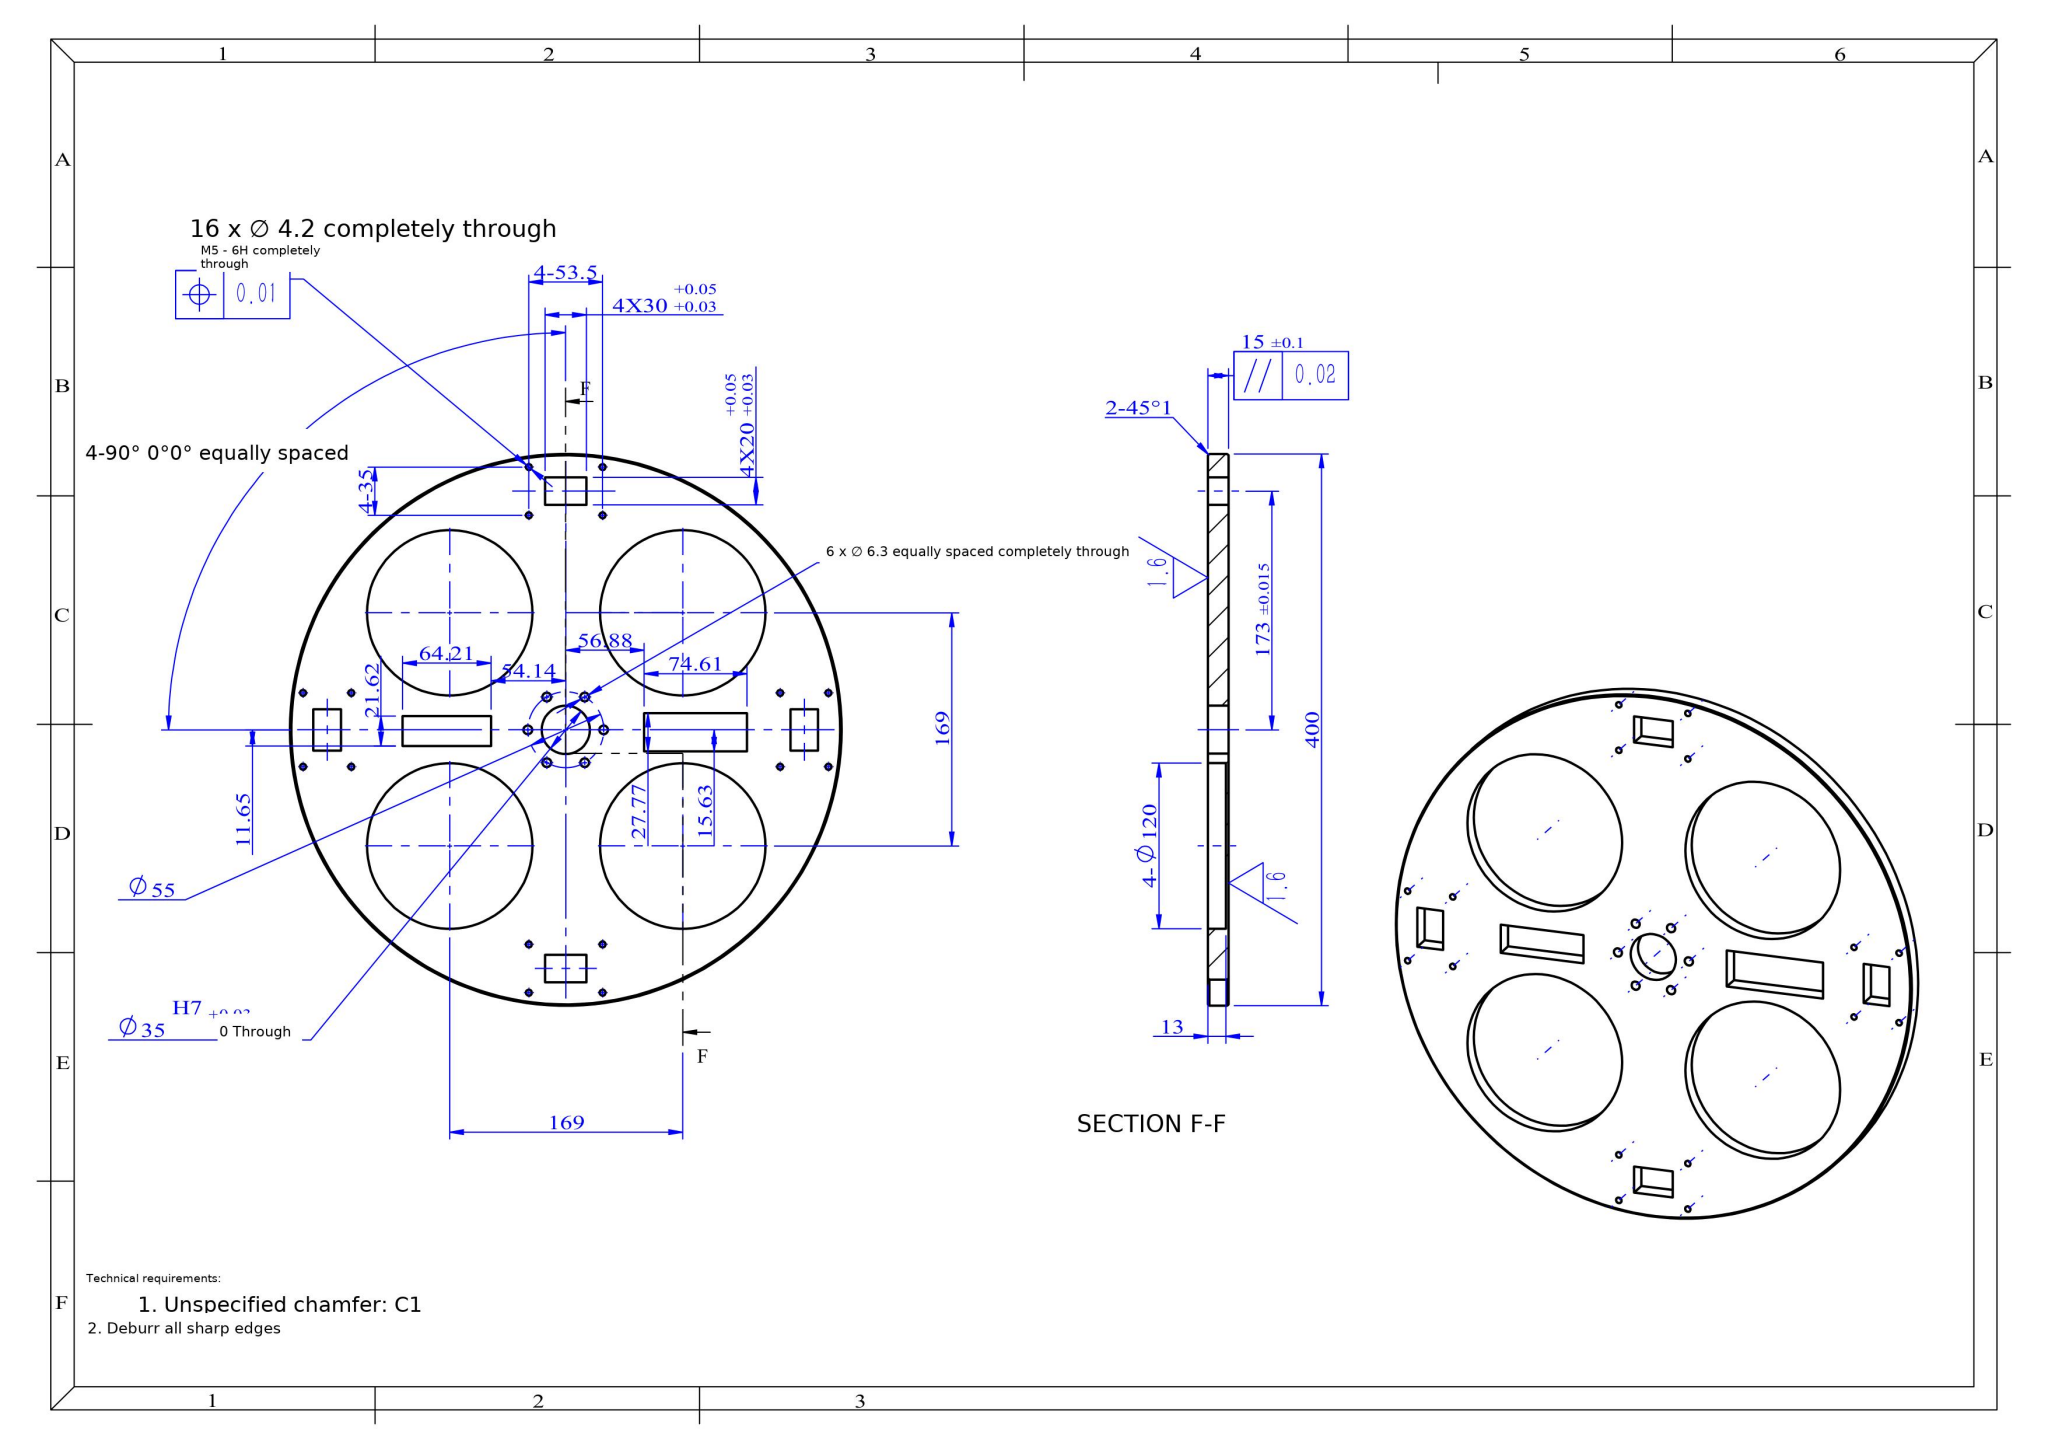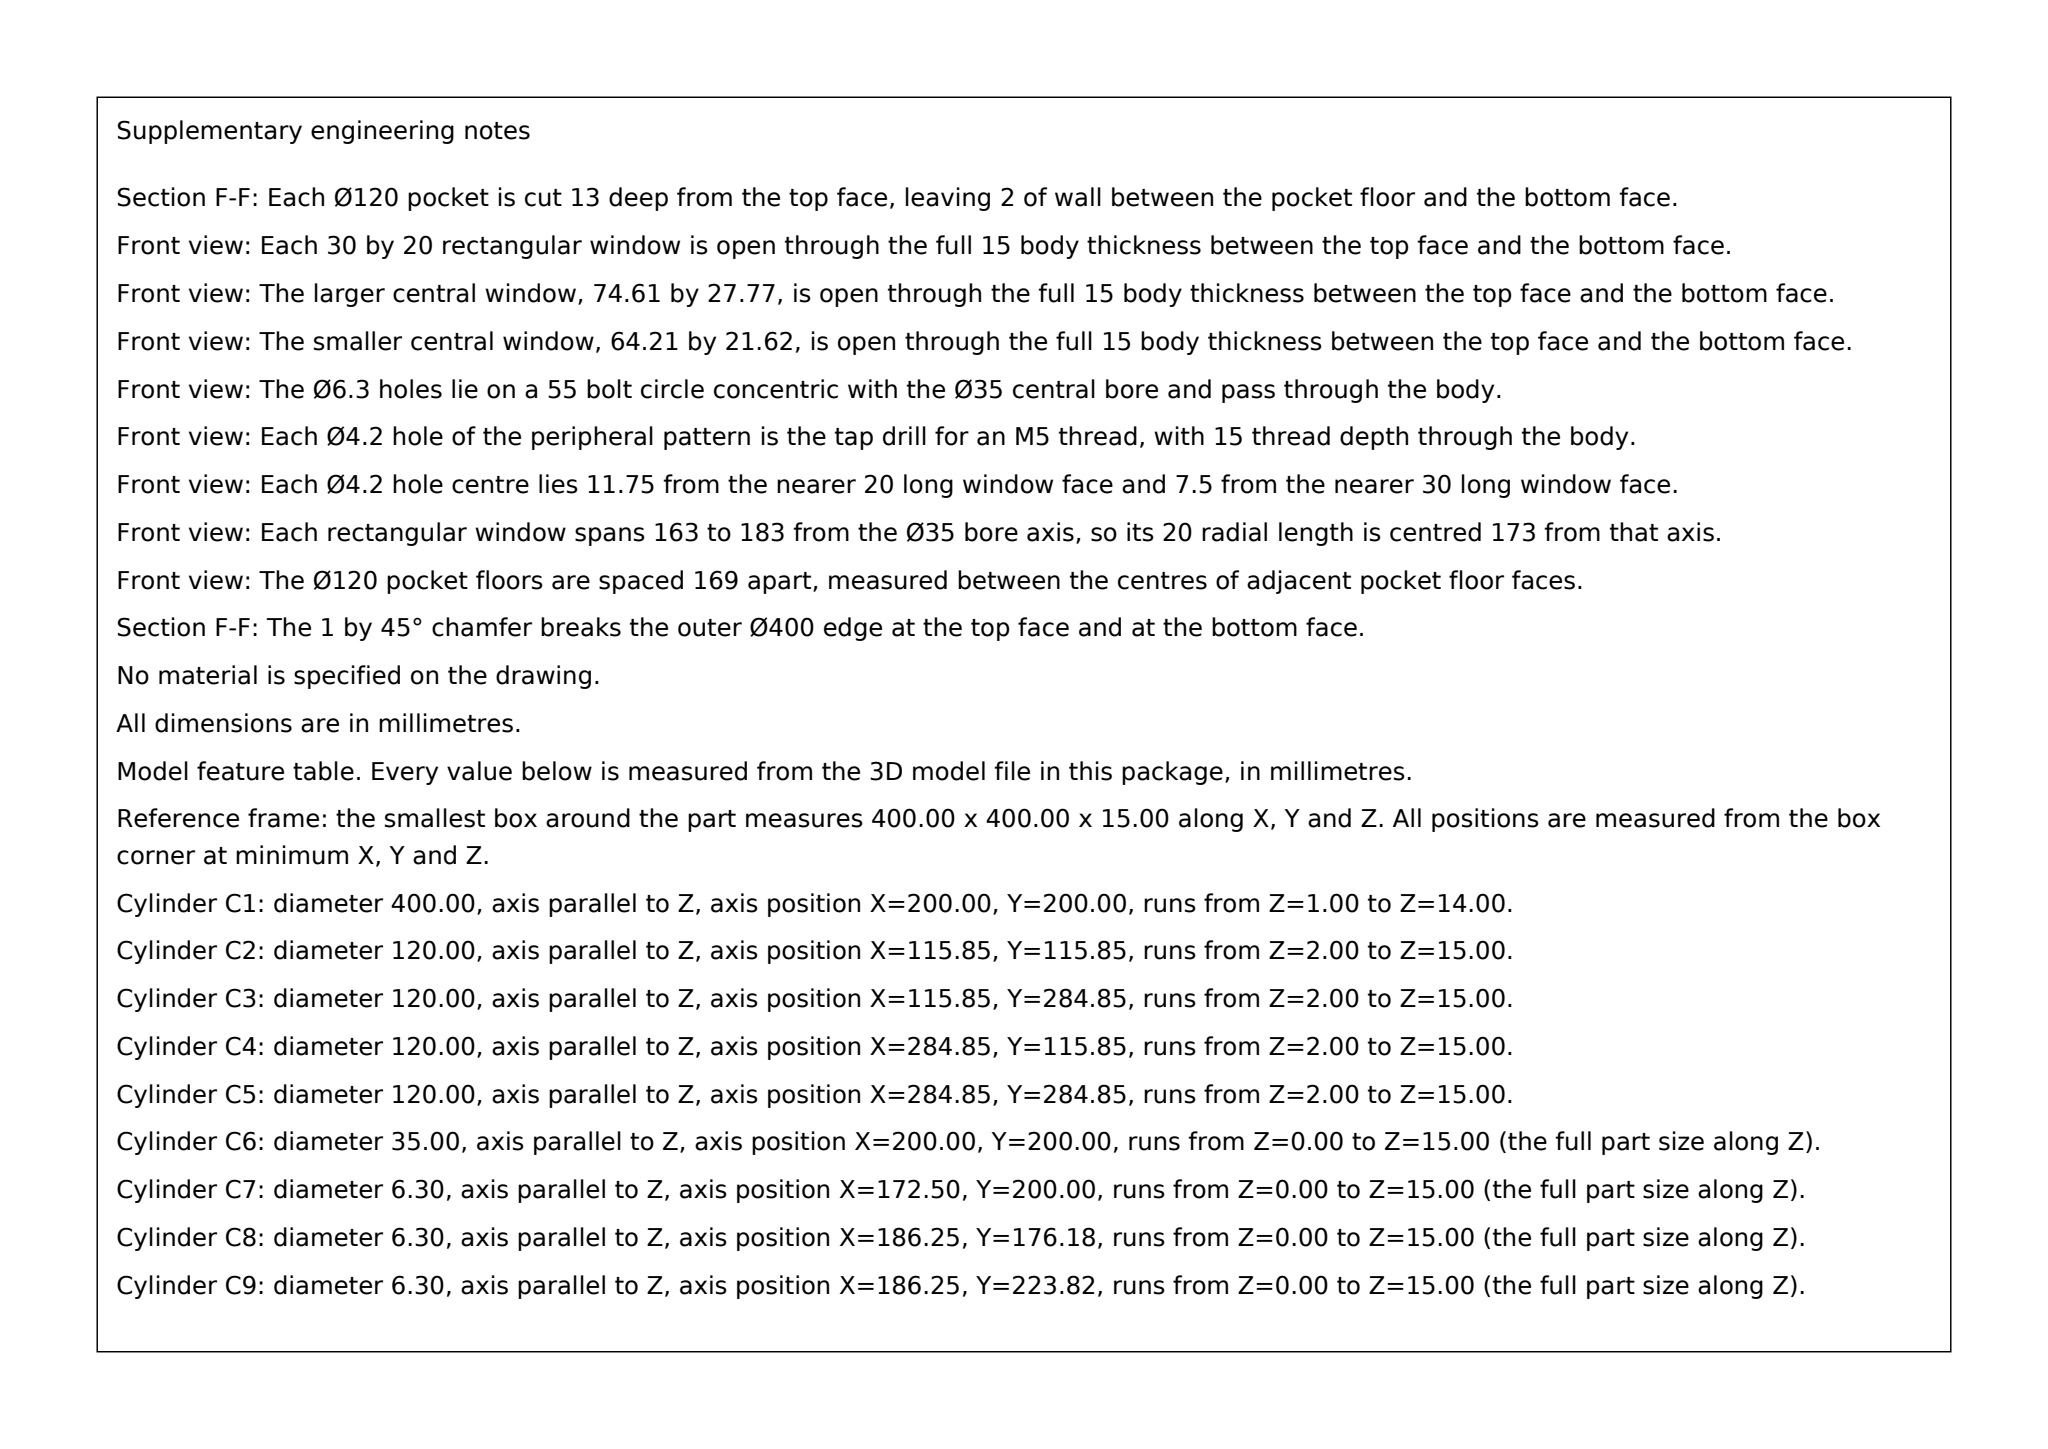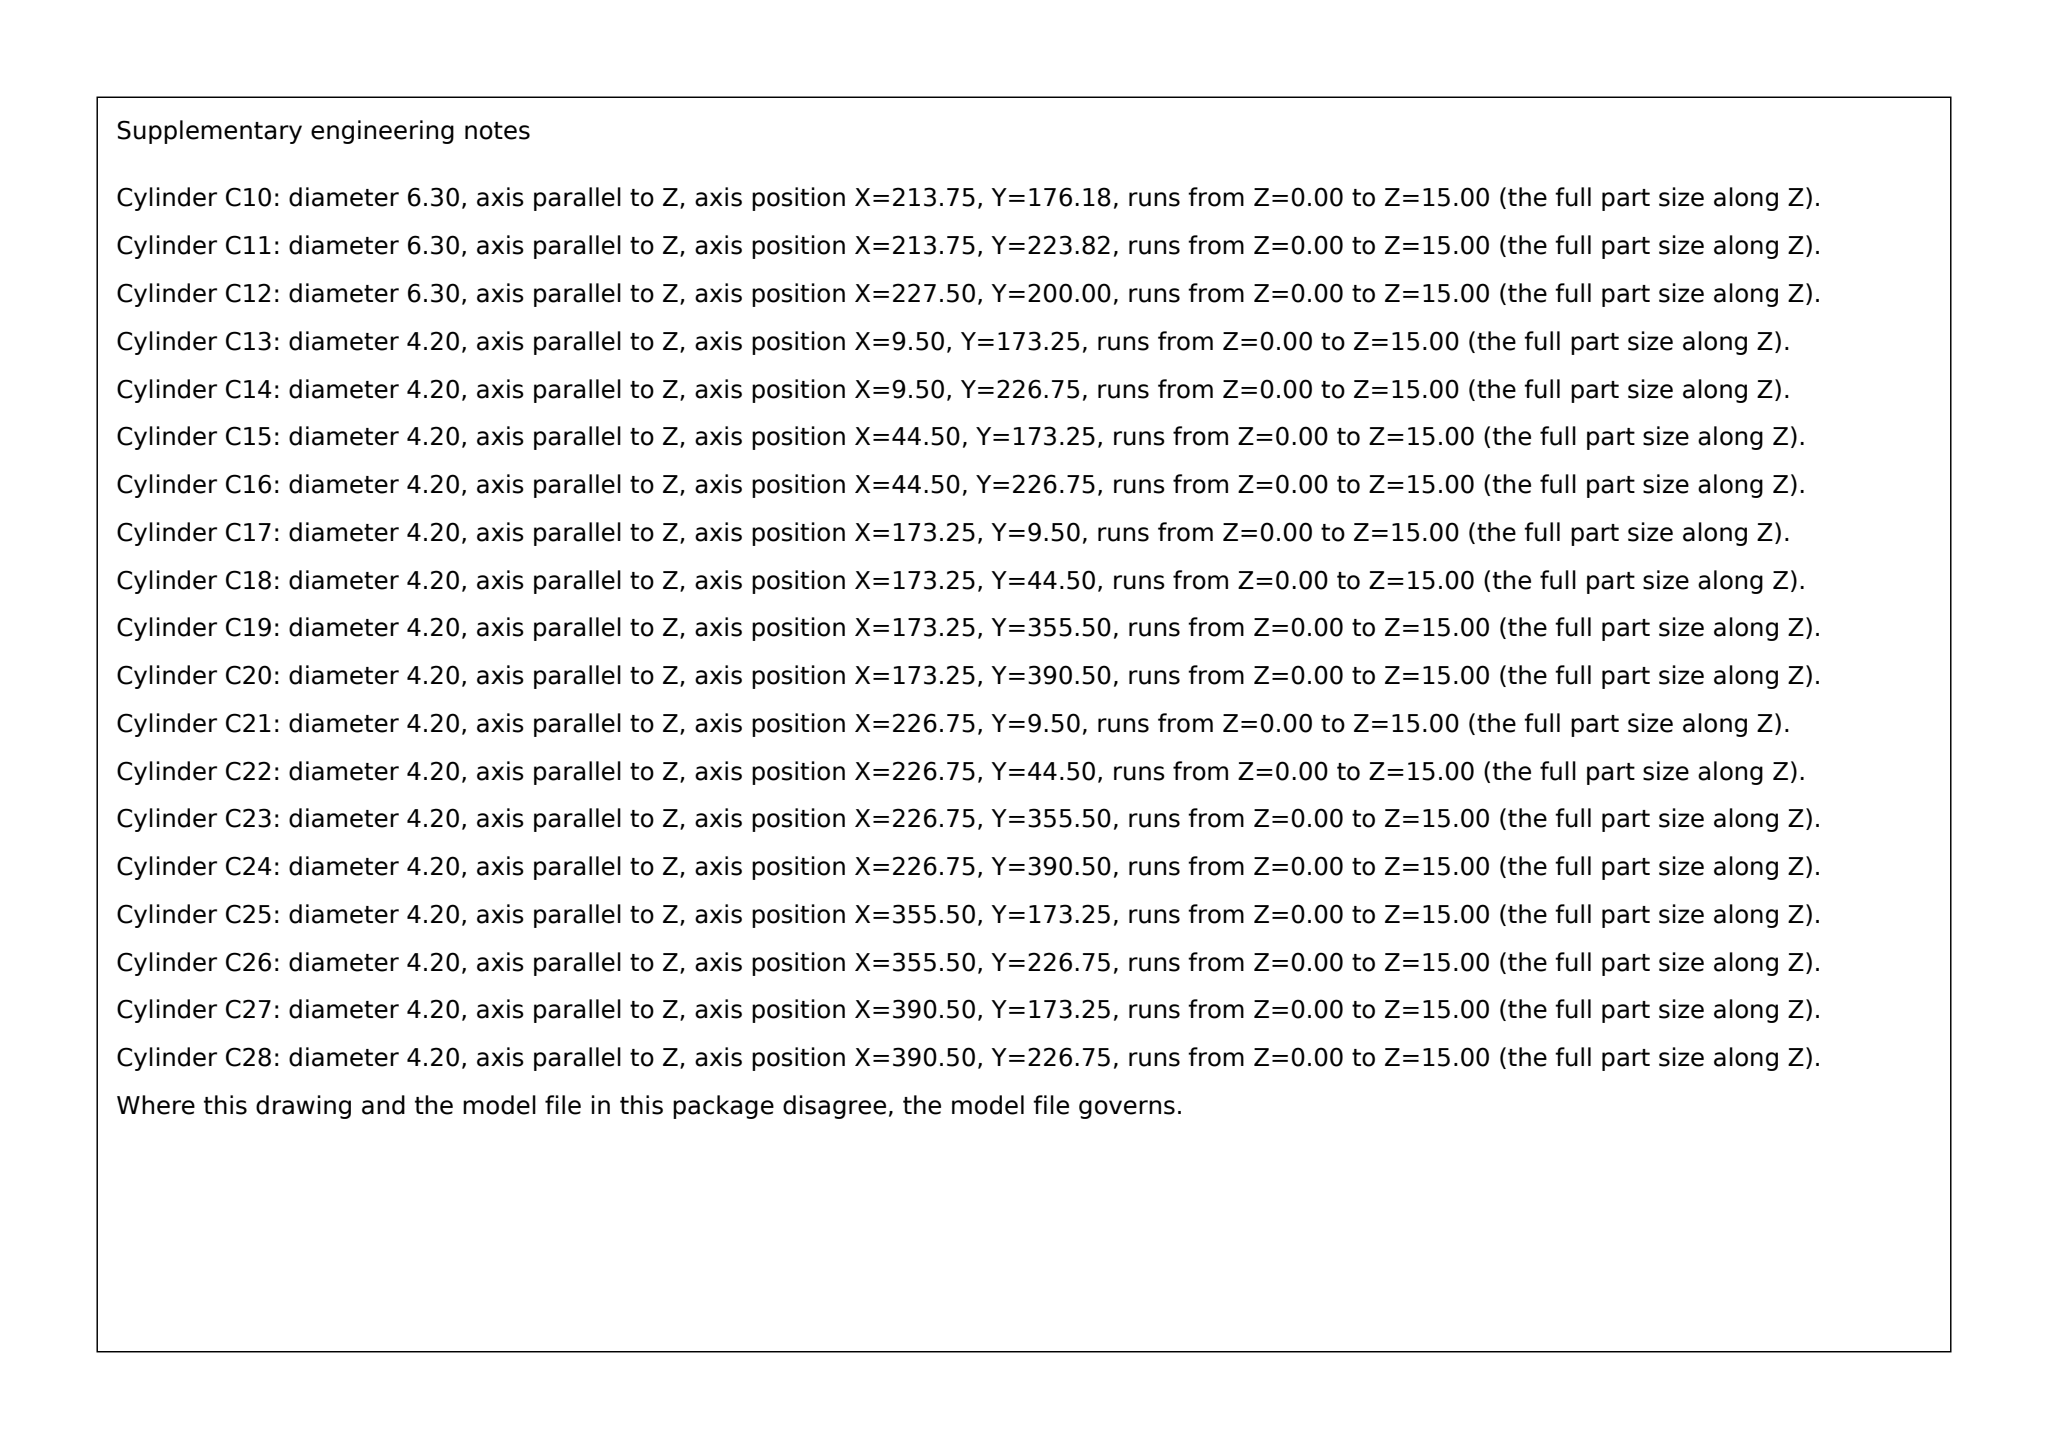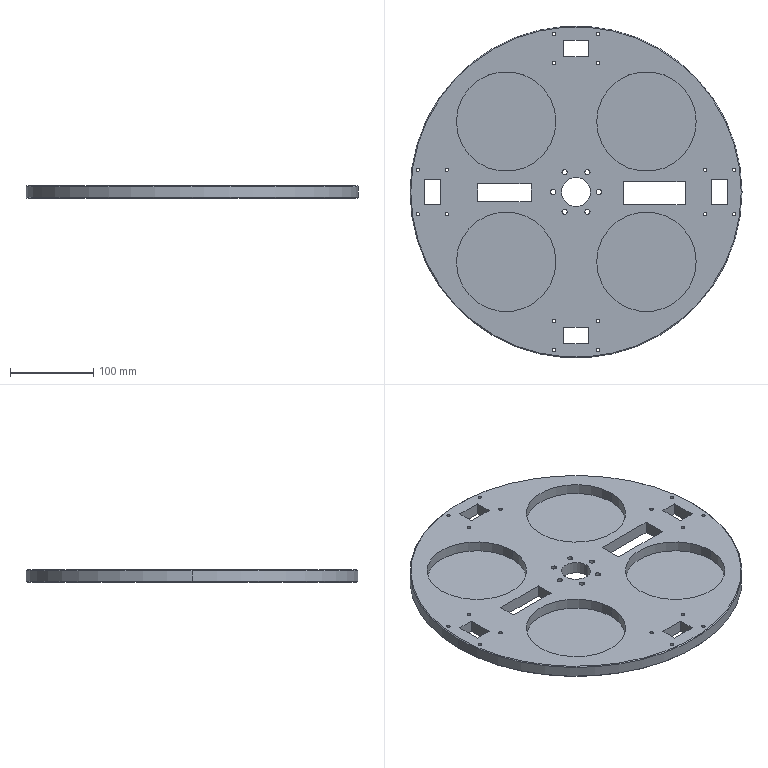Part | SolidWorks | mm | 1 solid | 90 faces | box 400 x 400 x 15 mm | volume 1187132 mm3 | cylinder 56 | plane 30 | cone 4 | commonest cylinder face diameters 4.2 x32 6.3 x12 120 x8 35 x2 400 x2
Drawing notes:
4X Ø120 POCKET 13 DP FROM TOP FACE, 2 THK FLOOR REMAINING | from the solid: cyl dia120 len13 at (115.85/284.85, 115.85/284.85); floor planes z=2 x4; plate thk 15
LH SLOT 64.21 X 21.62 THRU, 54.14 FROM CL, 11.65 BELOW CL | from the solid: x planes 81.65 & 145.86 (64.21); y planes 188.35 & 209.97 (21.62); CL at 200
RH SLOT 74.61 X 27.76 THRU, 56.88 FROM CL, 15.63 BELOW CL | from the solid: x planes 256.88 & 331.49 (74.61); y planes 184.37 & 212.13 (27.76); CL at 200
4X PERIPH SLOT 30 X 20 THRU, ON CL, 17 FROM Ø400 EDGE | from the solid: x/y planes 17 & 37 with 185 & 215 pairs; bbox 400x400
4X Ø120 PCKT PATTERN CTR: 0.35 +X, 0.35 +Y FROM Ø35 BORE CL | from the solid: Ø120 pockets at (115.85,115.85),(115.85,284.85),(284.85,115.85),(284.85,284.85); pattern ctr (200.35,200.35) vs Ø35 bore & 400 OD ctr (200,200); 169 spacing both axes
RH INTERNAL SLOT WIDTH 27.76 (SUPERSEDES 27.77) | from the solid: y-planes 184.37 & 212.13 bounding RH slot (x 215.0 to 256.88): 212.13-184.37 = 27.76
6X Ø6.3 ON Ø55 B.C.: 2 HOLES ON HORIZ CL, 60° EQL SP | from the solid: Ø6.3 holes at (172.5,200) & (227.5,200) = horizontal CL, R27.5; others (186.25,176.18),(186.25,223.82),(213.75,176.18),(213.75,223.82) = ±60° increments
Ø35 H7 BORE THRU (15 THK), CENTRED ON PLATE CL, 200 FROM EACH Ø400 EDGE | from the solid: cylinders: [35.0,"z",[200.0,200.0],15.0] ; bbox_xyz 400x400x15
16X Ø4.2 THRU, 4 GROUPS OF 4 AT 90° ABOUT CTR; EACH HOLE 26.75 EITHER SIDE OF CL AND 9.5 / 44.5 FROM Ø400 EDGE | from the solid: cylinders: sixteen 4.2 dia, z, length 15, at (9.5/44.5/355.5/390.5, 173.25/226.75) and (173.25/226.75, 9.5/44.5/355.5/390.5)
CHAMFER 1 X 45° ON Ø400 OD, BOTH FACES | from the solid: cones: [90.0 included, ref_dia 400.0] and [90.0, ref_dia 398.0]
LH AND RH INTERNAL SLOTS ARE 2X THRU, FULL 15 THK, NO FLOOR | from the solid: bbox_xyz z=15 with slot wall axis_planes x 81.65/145.86 and x 256.88/331.49 and no z=2 floor plane at slots
Ø35 THRU BORE, CENTERED ON PLATE: 200 FROM EACH Ø400 EDGE (ON BOTH CL), FULL 15 THK | from the solid: cylinder dia 35, axis z, pos (200,200), length 15 = full bbox z
2X CHAMFER 1 X 45° ON Ø400 OUTSIDE EDGE, BOTH FACES | from the solid: cones 90.0 included angle at ref dia 400 and 398 (1 mm radial run-out)
4X PERIPHERAL SLOTS 30 WIDE X 20 DEEP, THRU 15 THK, EQUALLY SPACED 90° ON THE TWO CENTERLINES | from the solid: axis_planes x=17/37 and x=363/383; y=17/37 and y=363/383 (30 wide between 185/215, 20 deep from edge)
BOTH INTERNAL RECTANGULAR SLOTS (LH AND RH) ARE THRU, FULL 15 PLATE THK | from the solid: slot faces x=81.65/145.86 and x=256.88/331.49 with bbox z=15 (no floor plane at z=2 within slots)
Ø35 THRU BORE, CENTRED AT X200 Y200 FROM MIN CORNER OF 400 X 400 PLATE | from the solid: cylinders: [35.0,"z",[200.0,200.0],15.0]
16X Ø4.2 THRU (4 GROUPS OF 4): CENTRES AT X=9.5/44.5 AND X=355.5/390.5 WITH Y=173.25/226.75, AND Y=9.5/44.5 AND Y=355.5/390.5 WITH X=173.25/226.75, FROM MIN CORNER | from the solid: cylinders: 16 off [4.2,"z",...,15.0]
2X CHAMFER 1 X 45° ON Ø400 OD, BOTH FACES | from the solid: cones: [90.0,400.0,2] and [90.0,398.0,2]
ALL Ø4.2, Ø6.3, Ø35 HOLES AND ALL SLOTS THRU FULL 15 THK PLATE | from the solid: cylinder lengths 15.0 and bbox_xyz z = 15.0
4X Ø120 POCKET CENTRES AT X/Y 115.85 AND 284.85 FROM MIN CORNER, 13 DEEP (2 THK FLOOR) | from the solid: cylinders: [120.0,"z",[115.85/284.85,115.85/284.85],13.0]; plane z=2.0 (4)
build123d program:
from build123d import *

# Parameters (mm, degrees)
SKETCH1_R                  = 200
BOSS_EXTRUDE1_DEPTH        = 15
SKETCH2_W                  = 30
SKETCH2_H                  = 20
CUT_EXTRUDE1_DEPTH         = 284.24
CIRPATTERN1_COUNT          = 4
M5_TAPPED_HOLE1_D          = 4.2
CIRPATTERN2_COUNT          = 4
CHAMFER1_SIZE              = 1
SKETCH5_R                  = 17.5
CUT_EXTRUDE2_DEPTH         = 284.24
F_6_3_6_3_DIAMETER_HOLE1_D = 6.3
SKETCH9_R                  = 60
CUT_EXTRUDE4_DEPTH         = 13
SKETCH10_W                 = 64.215
SKETCH10_H                 = 21.62
SKETCH10_W_2               = 74.607
SKETCH10_H_2               = 27.769
CUT_EXTRUDE5_DEPTH         = 108


with BuildPart() as part:
    # Sketch1 → Boss-Extrude1 (new body)
    with BuildSketch(Plane.XY):
        Circle(SKETCH1_R)
    extrude(amount=BOSS_EXTRUDE1_DEPTH)

    # Sketch2 → Cut-Extrude1 (cut, through all)
    with BuildSketch(Plane.XY.offset(15)):
        with Locations((0, 173)):
            Rectangle(SKETCH2_W, SKETCH2_H)
    cut_extrude1 = extrude(amount=-CUT_EXTRUDE1_DEPTH, mode=Mode.SUBTRACT)

    # CirPattern1: Cut-Extrude1 ×4 about axis
    cirpattern1_axis = Axis((0, 0, 0), (0, 0, 1))
    for i in range(1, CIRPATTERN1_COUNT):
        add(cut_extrude1.rotate(cirpattern1_axis, i * 360 / CIRPATTERN1_COUNT), mode=Mode.SUBTRACT)

    # M5 Tapped Hole1 (through all)
    with Locations(Plane(origin=(0, 0, 0), x_dir=(-1, 0, 0), z_dir=(0, 0, -1))):
        with Locations((-26.75, -155.5), (-26.75, -190.5), (26.75, -155.5), (26.75, -190.5)):
            m5_tapped_hole1 = Hole(M5_TAPPED_HOLE1_D / 2)

    # CirPattern2: M5 Tapped Hole1 ×4 about axis
    cirpattern2_axis = Axis((0, 0, 0), (0, 0, 1))
    for i in range(1, CIRPATTERN2_COUNT):
        add(m5_tapped_hole1.rotate(cirpattern2_axis, i * 360 / CIRPATTERN2_COUNT), mode=Mode.SUBTRACT)

    # Chamfer1
    chamfer1_edges = [part.edges().sort_by_distance(p)[0] for p in [
        (-200, 0, 0),
        (-200, 0, 15),
    ]]
    chamfer(chamfer1_edges, length=CHAMFER1_SIZE)

    # Sketch5 → Cut-Extrude2 (cut, through all)
    with BuildSketch(Plane(origin=(0, 0, 0), x_dir=(-1, 0, 0), z_dir=(0, 0, -1))):
        Circle(SKETCH5_R)
    extrude(amount=-CUT_EXTRUDE2_DEPTH, mode=Mode.SUBTRACT)

    # 6.3 _6.3_ Diameter Hole1 (through all)
    with Locations(Plane(origin=(0, 0, 0), x_dir=(-1, 0, 0), z_dir=(0, 0, -1))):
        with Locations((-13.75, 23.816), (13.75, 23.816), (27.5, 0), (13.75, -23.816), (-13.75, -23.816), (-27.5, 0)):
            Hole(F_6_3_6_3_DIAMETER_HOLE1_D / 2)

    # Sketch9 → Cut-Extrude4 (cut)
    with BuildSketch(Plane.XY.offset(15)):
        with Locations((84.853, 84.853)):
            Circle(SKETCH9_R)
        with Locations((84.853, -84.147)):
            Circle(SKETCH9_R)
        with Locations((-84.147, -84.147)):
            Circle(SKETCH9_R)
        with Locations((-84.147, 84.853)):
            Circle(SKETCH9_R)
    extrude(amount=-CUT_EXTRUDE4_DEPTH, mode=Mode.SUBTRACT)

    # Sketch10 → Cut-Extrude5 (cut)
    with BuildSketch(Plane.XY.offset(15)):
        with Locations((-86.246, -0.839)):
            Rectangle(SKETCH10_W, SKETCH10_H)
        with Locations((94.185, -1.75)):
            Rectangle(SKETCH10_W_2, SKETCH10_H_2)
    extrude(amount=-CUT_EXTRUDE5_DEPTH, mode=Mode.SUBTRACT)


solid = part.part